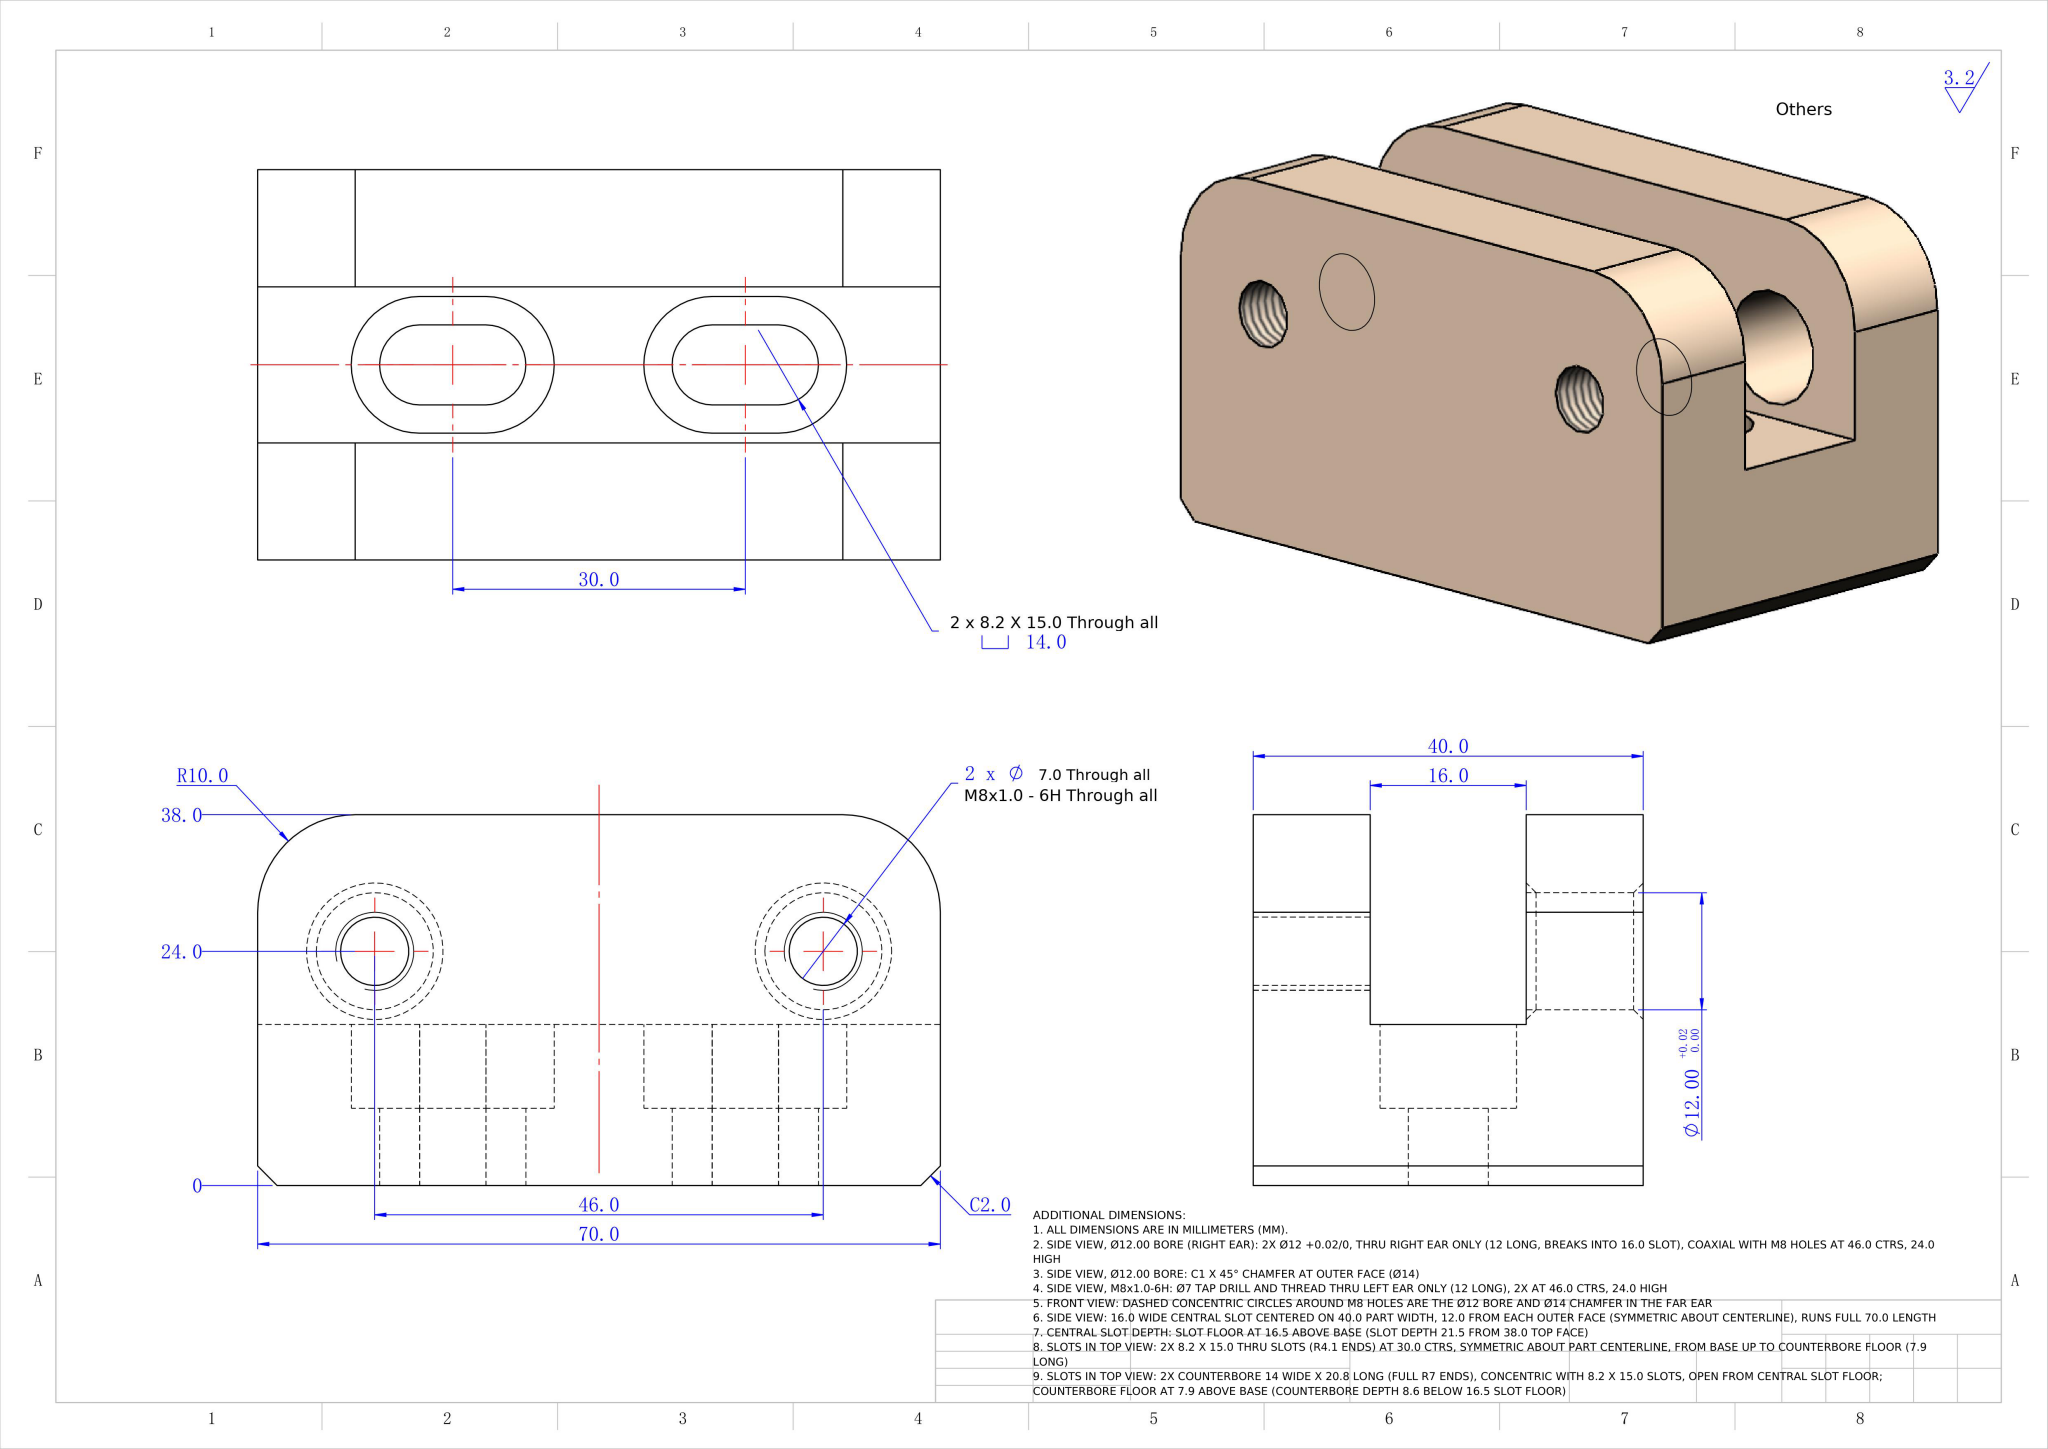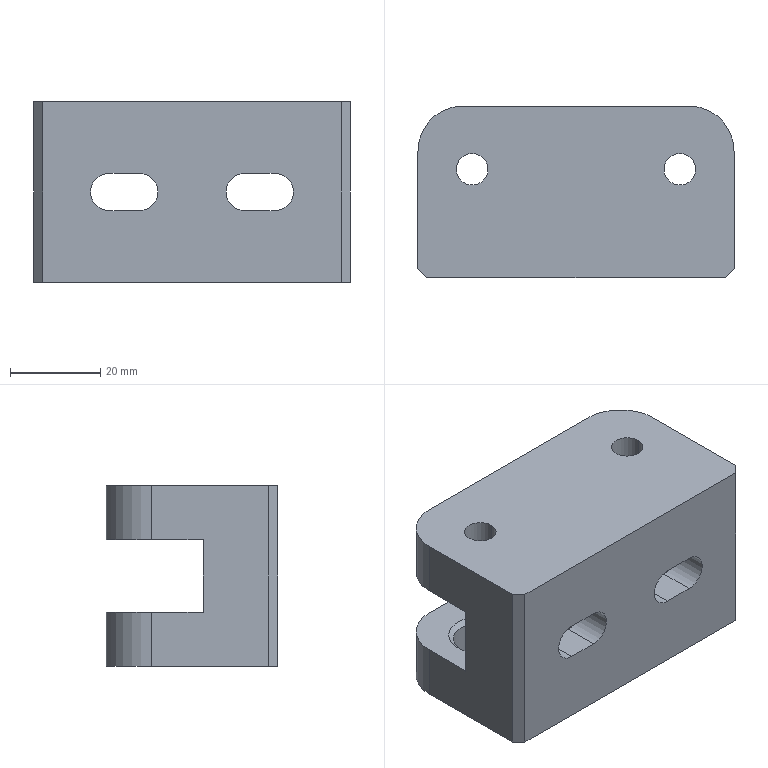Part | NX | mm | 1 solid | 48 faces | box 70 x 38 x 40 mm | volume 71432 mm3 | plane 22 | cylinder 20 | cone 6 | commonest cylinder face diameters 7 x4 12 x4 20 x4 8.2 x4 14 x4